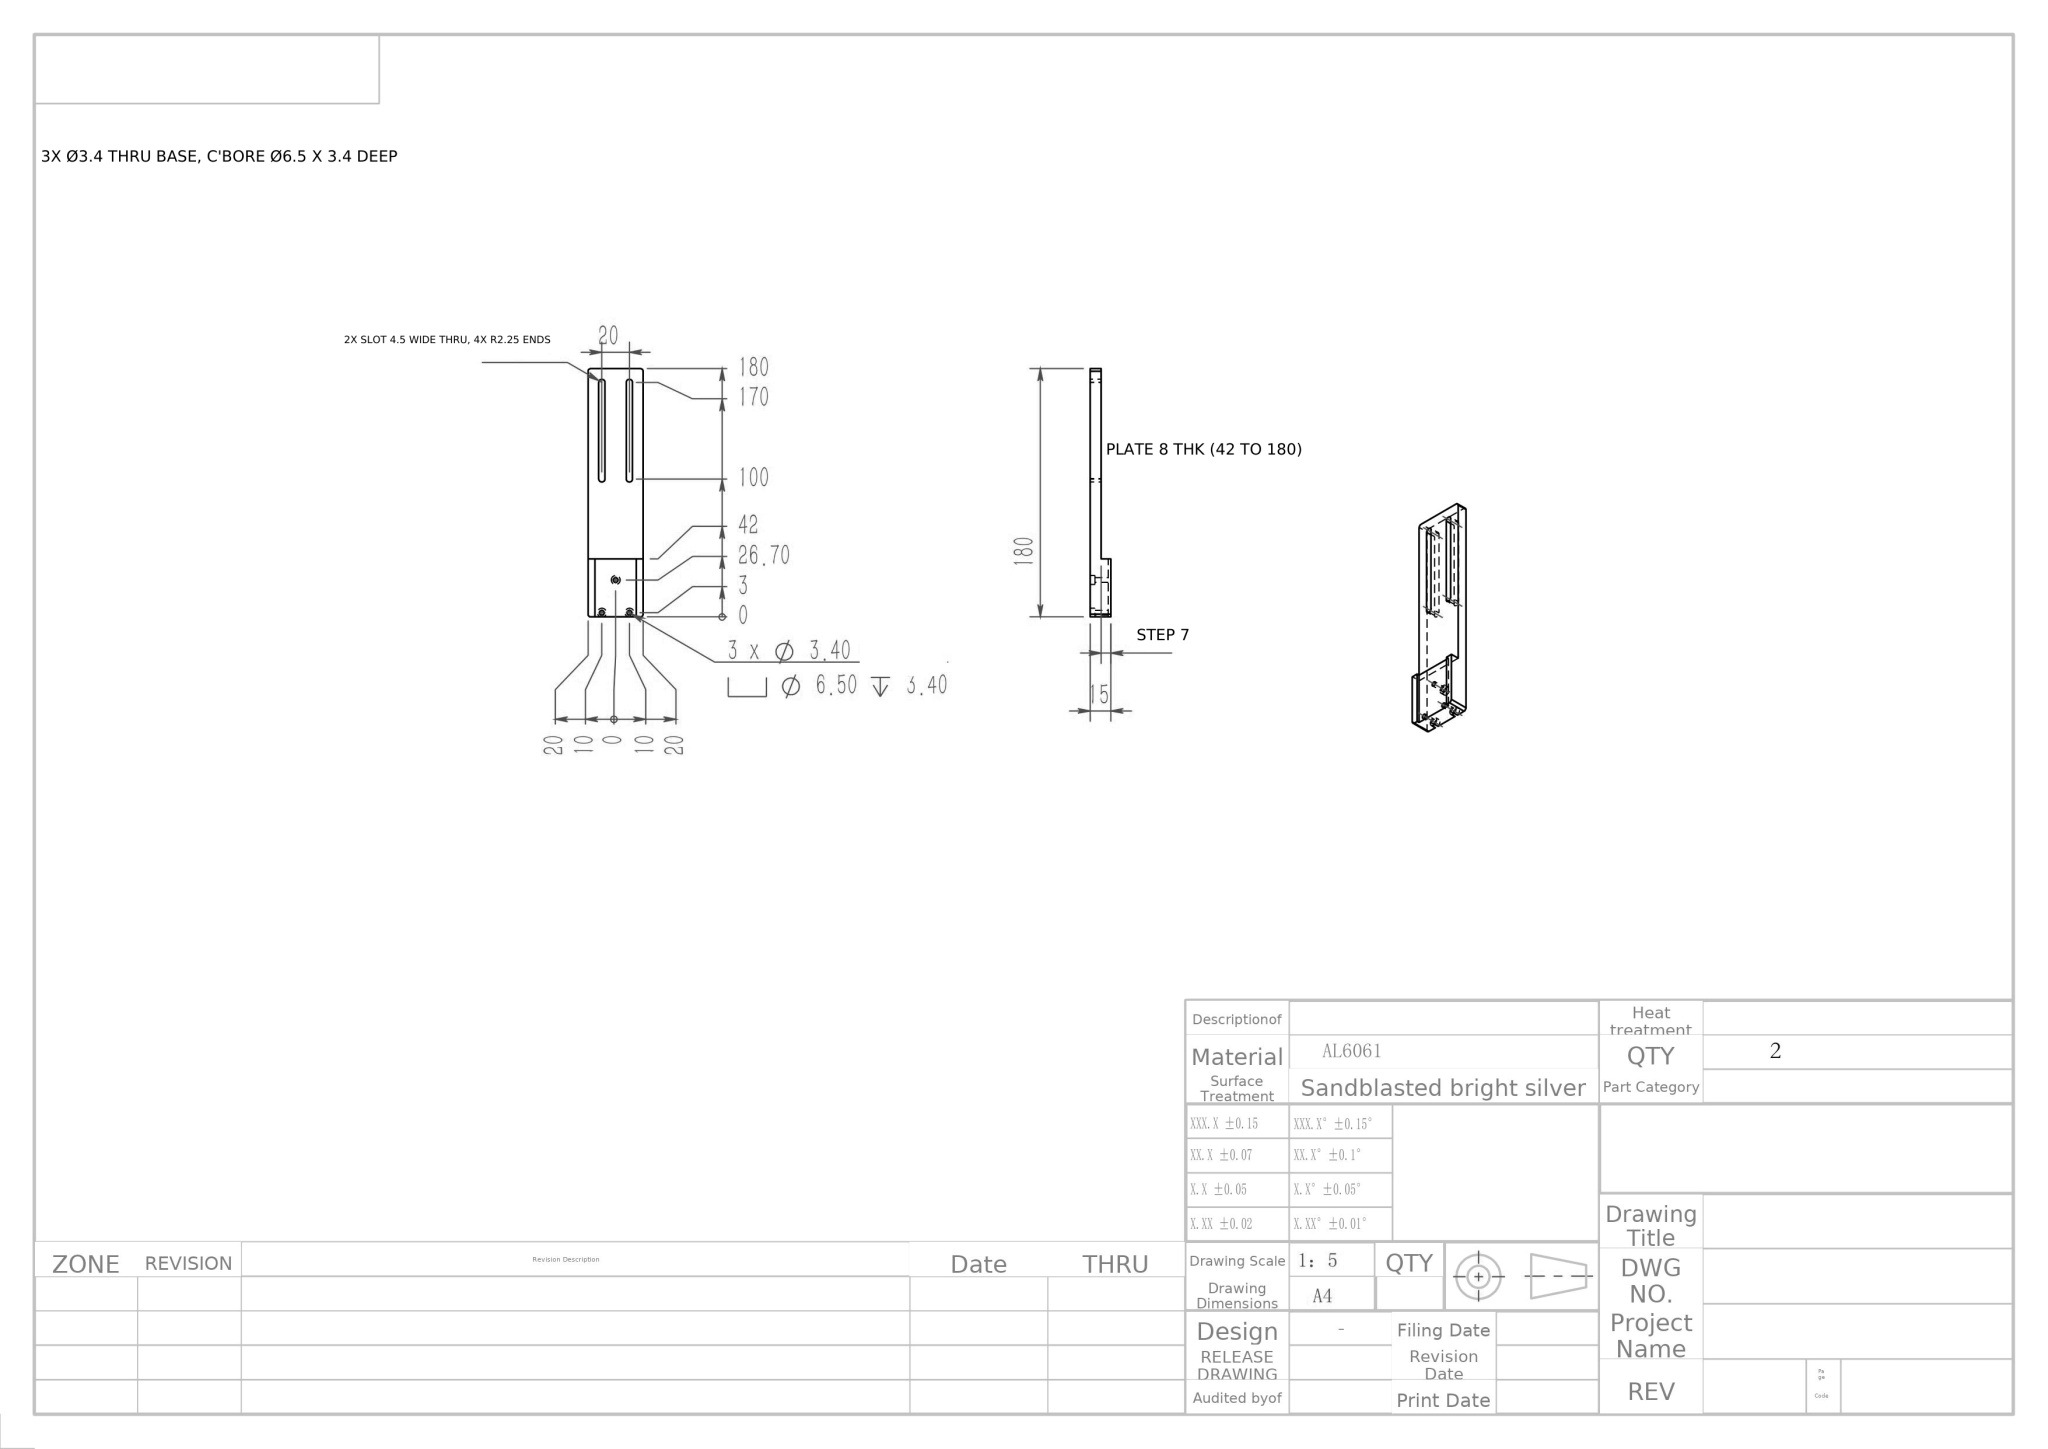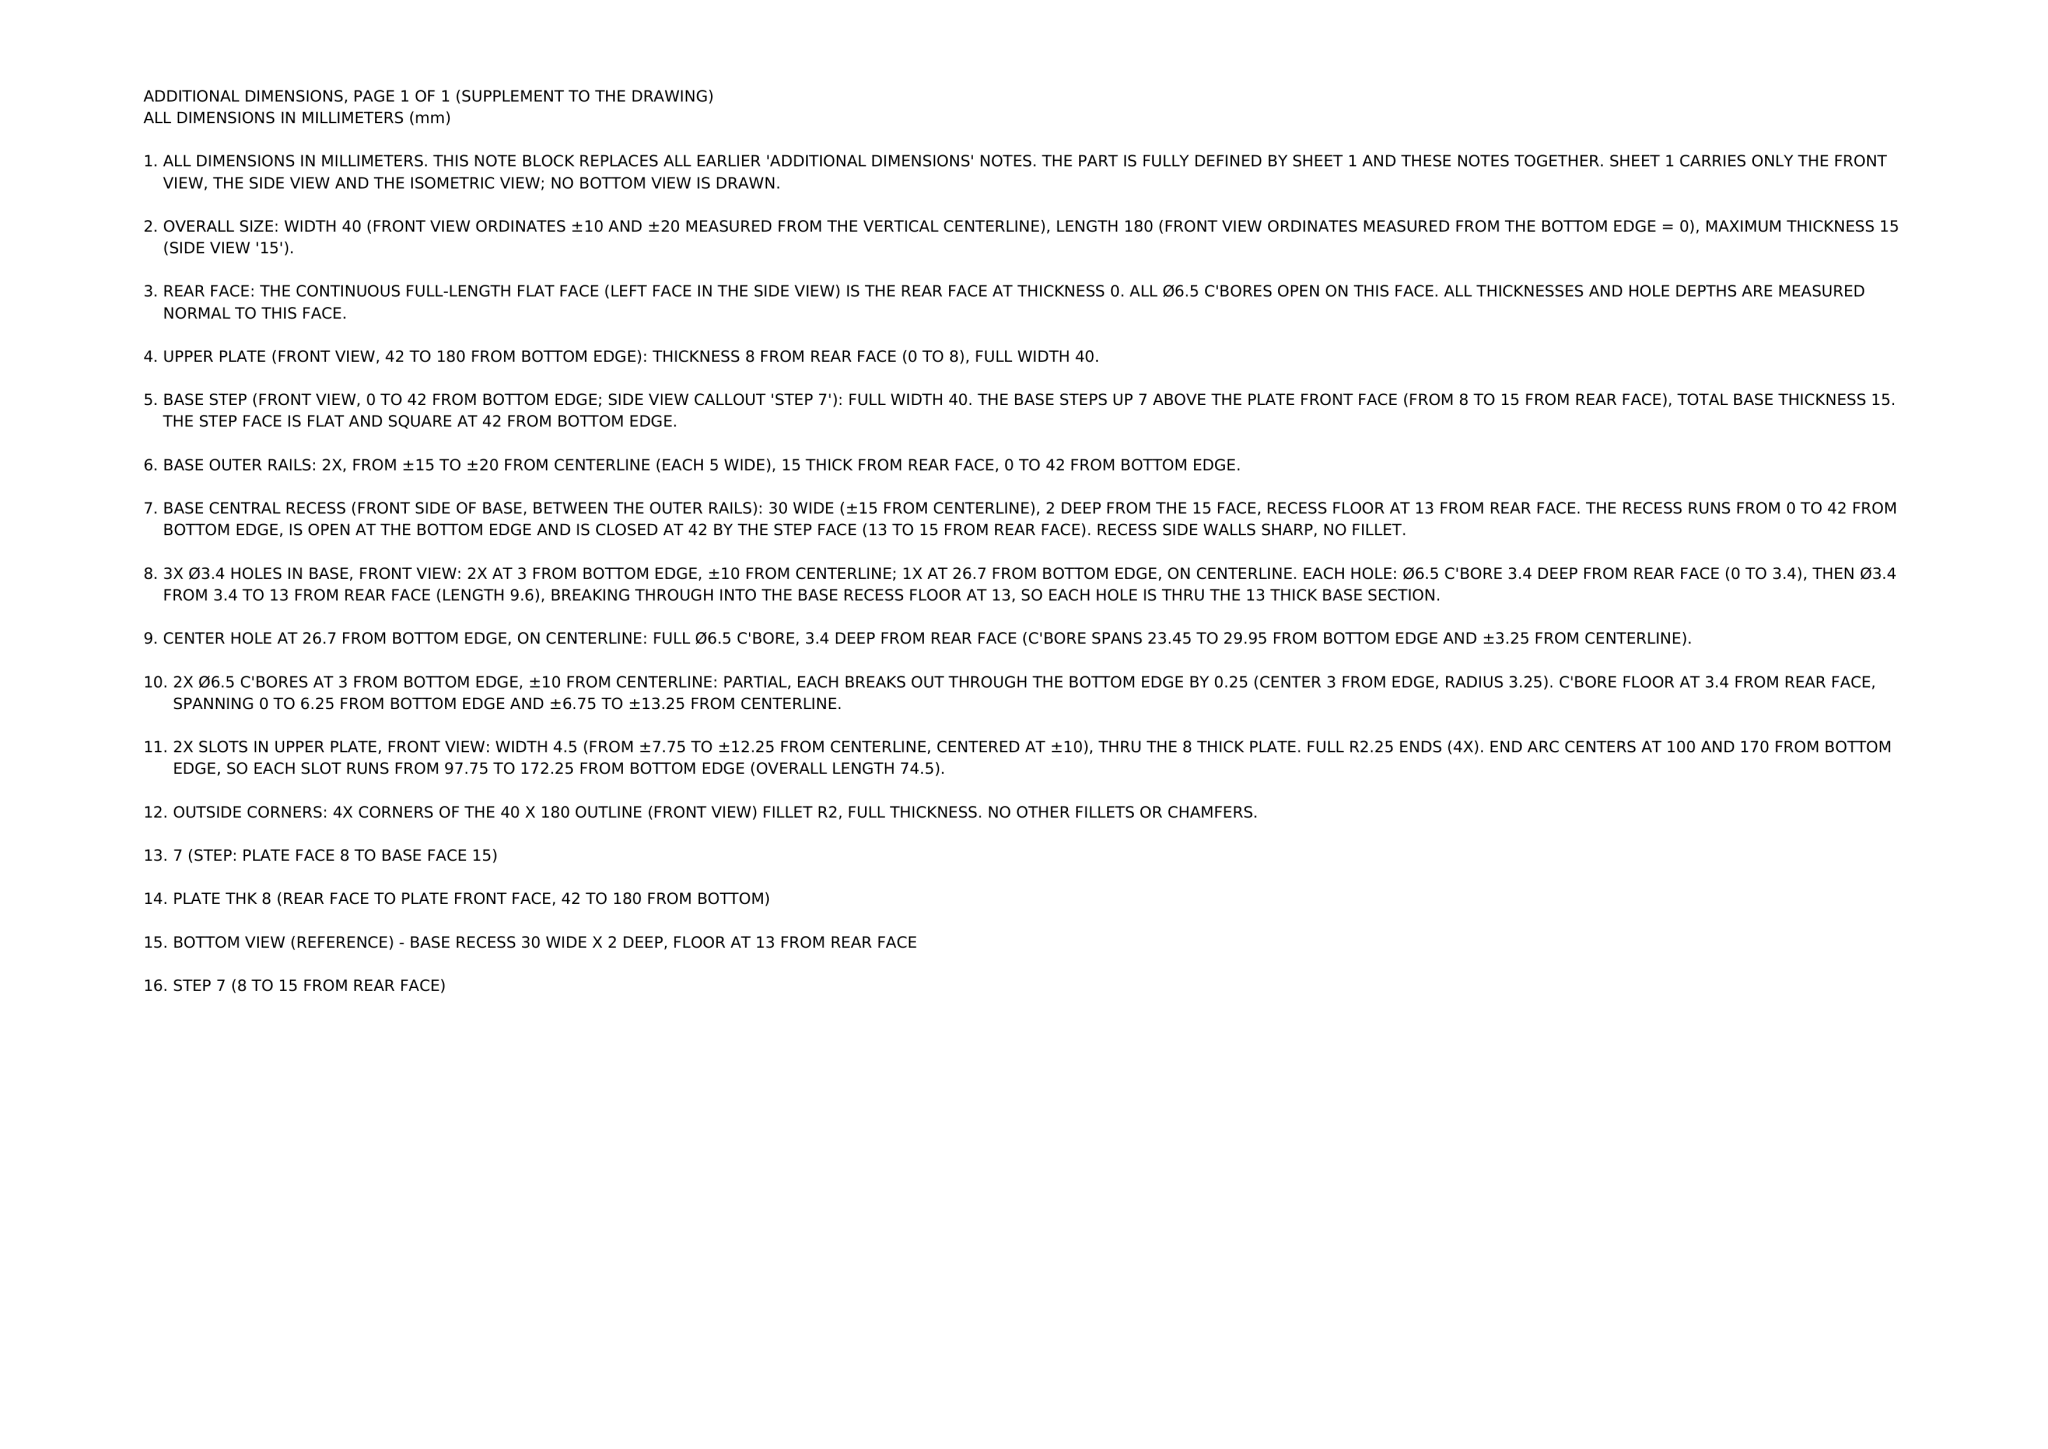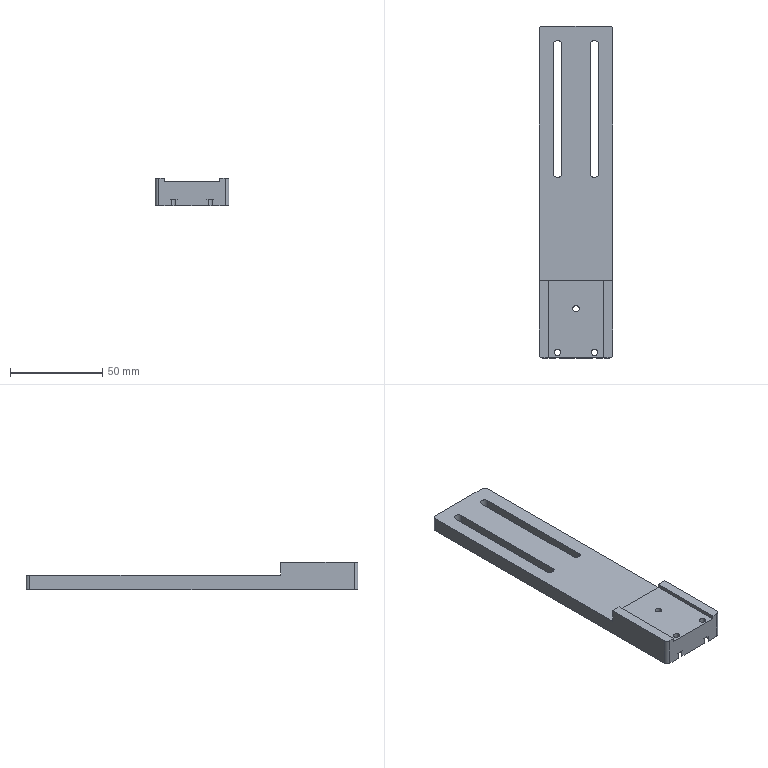Part | NX | mm | 1 solid | 41 faces | box 40 x 180 x 15 mm | volume 60909 mm3 | cylinder 22 | plane 19 | commonest cylinder face diameters 6.5 x8 3.4 x6 4 x4 4.5 x4